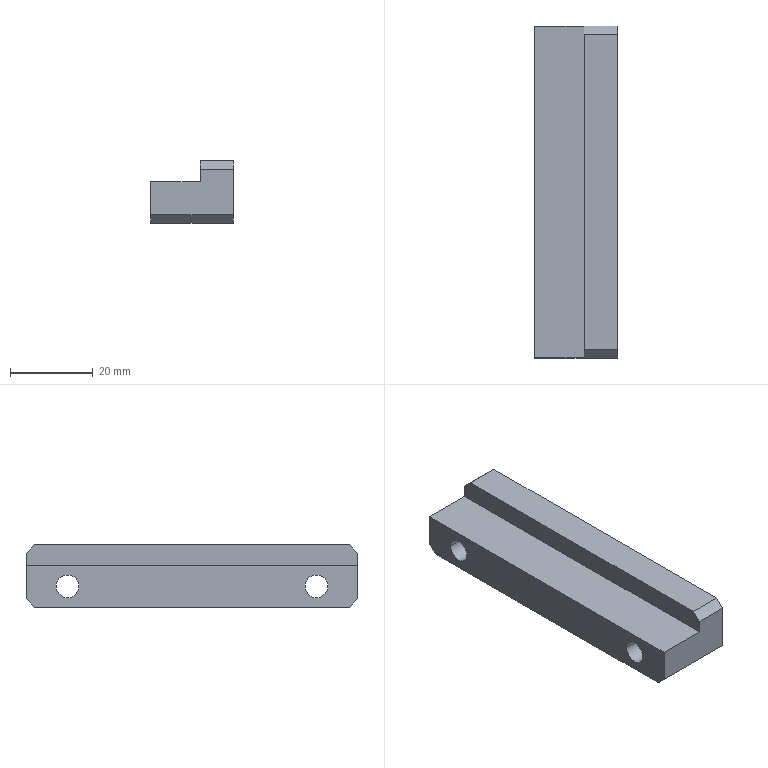Component | SolidWorks | ClampingAssembly-1_A84-2 | 1 solid | 24 faces | box 20 x 80 x 15 mm | volume 17417 mm3 | plane 18 | cylinder 6 | commonest cylinder face diameters 5.5 x4 10 x2 | material S136
build123d program:
from build123d import *

# Parameters (mm, degrees)
SKETCH1_W                  = 80
SKETCH1_H                  = 15
BOSS_EXTRUDE1_DEPTH        = 10
SKETCH2_W                  = 12
SKETCH2_H                  = 5
CUT_EXTRUDE1_DEPTH         = 81.971
CHAMFER1_SIZE              = 2
F_5_5_5_5_DIAMETER_HOLE1_D = 5.5
CUT_EXTRUDE2_DEPTH         = 5.5


with BuildPart() as part:
    # Sketch1 → Boss-Extrude1 (new, symmetric)
    with BuildSketch(Plane(origin=(0, 0, 0), x_dir=(0, 0, -1), z_dir=(1, 0, 0))):
        Rectangle(SKETCH1_W, SKETCH1_H)
    extrude(amount=BOSS_EXTRUDE1_DEPTH, both=True)

    # Sketch2 → Cut-Extrude1 (cut, through all)
    with BuildSketch(Plane(origin=(0, 0, -40), x_dir=(-1, 0, 0), z_dir=(0, 0, -1))):
        with Locations((4, -5)):
            Rectangle(SKETCH2_W, SKETCH2_H)
    extrude(amount=-CUT_EXTRUDE1_DEPTH, mode=Mode.SUBTRACT)

    # Chamfer1
    chamfer1_edges = [part.edges().sort_by_distance(p)[0] for p in [
        (6, -7.5, -40),
        (6, -7.5, 40),
        (0, 7.5, 40),
        (0, 7.5, -40),
    ]]
    chamfer(chamfer1_edges, length=CHAMFER1_SIZE)

    # 5.5 _5.5_ Diameter Hole1 (through all)
    with Locations(Plane(origin=(10, 0, 0), x_dir=(0, 0, -1), z_dir=(1, 0, 0))):
        with Locations((-30, 2.5), (30, 2.5)):
            Hole(F_5_5_5_5_DIAMETER_HOLE1_D / 2)

    # Sketch7 → Cut-Extrude2 (cut)
    with BuildSketch(Plane(origin=(10, 0, 0), x_dir=(0, 0, -1), z_dir=(1, 0, 0))):
        with BuildLine():
            Line((-35, 2.5), (-35, 7.5))
            ThreePointArc((-35, 7.5), (-30, 12.5), (-25, 7.5))
            Line((-25, 7.5), (-25, 2.5))
            ThreePointArc((-25, 2.5), (-30, -2.5), (-35, 2.5))
        make_face()
        with BuildLine():
            Line((25, 2.5), (25, 7.5))
            ThreePointArc((25, 7.5), (30, 12.5), (35, 7.5))
            Line((35, 7.5), (35, 2.5))
            ThreePointArc((35, 2.5), (30, -2.5), (25, 2.5))
        make_face()
    extrude(amount=-CUT_EXTRUDE2_DEPTH, mode=Mode.SUBTRACT)


solid = part.part

# Placed as in the assembly
solid = solid.moved(Location((-4.551, 48.036, -72), (-90, 0, 0)))
STEP:
#1=COLOUR_RGB('',0.7922,0.8196,0.9333);
#2=FILL_AREA_STYLE_COLOUR('',#1);
#3=FILL_AREA_STYLE('',(#2));
#4=SURFACE_STYLE_FILL_AREA(#3);
#5=SURFACE_SIDE_STYLE('',(#4));
#6=SURFACE_STYLE_USAGE(.BOTH.,#5);
#7=PRESENTATION_STYLE_ASSIGNMENT((#6));
#8=CARTESIAN_POINT('',(-0.5729,3.181,-2.933));
#9=VERTEX_POINT('',#8);
#10=CARTESIAN_POINT('',(-0.5729,2.964,-2.933));
#11=VERTEX_POINT('',#10);
#12=CARTESIAN_POINT('',(-0.5729,3.072,-2.933));
#13=DIRECTION('',(1.,-0.,-0.));
#14=DIRECTION('',(0.,-1.,0.));
#15=AXIS2_PLACEMENT_3D('',#12,#13,#14);
#16=CIRCLE('',#15,0.1083);
#17=EDGE_CURVE('',#9,#11,#16,.T.);
#18=ORIENTED_EDGE('',*,*,#17,.F.);
#19=CARTESIAN_POINT('',(-0.001999,3.181,-2.933));
#20=VERTEX_POINT('',#19);
#21=CARTESIAN_POINT('',(0.2145,3.181,-2.933));
#22=DIRECTION('',(1.,-0.,-0.));
#23=VECTOR('',#22,39.37);
#24=LINE('',#21,#23);
#25=EDGE_CURVE('',#9,#20,#24,.T.);
#26=ORIENTED_EDGE('',*,*,#25,.T.);
#27=CARTESIAN_POINT('',(-0.001999,2.964,-2.933));
#28=VERTEX_POINT('',#27);
#29=CARTESIAN_POINT('',(-0.001999,3.072,-2.933));
#30=DIRECTION('',(-1.,0.,0.));
#31=DIRECTION('',(-0.,-1.,0.));
#32=AXIS2_PLACEMENT_3D('',#29,#30,#31);
#33=CIRCLE('',#32,0.1083);
#34=EDGE_CURVE('',#28,#20,#33,.T.);
#35=ORIENTED_EDGE('',*,*,#34,.F.);
#36=CARTESIAN_POINT('',(0.2145,2.964,-2.933));
#37=DIRECTION('',(1.,-0.,-0.));
#38=VECTOR('',#37,39.37);
#39=LINE('',#36,#38);
#40=EDGE_CURVE('',#11,#28,#39,.T.);
#41=ORIENTED_EDGE('',*,*,#40,.F.);
#42=EDGE_LOOP('',(#18,#26,#35,#41));
#43=FACE_OUTER_BOUND('',#42,.T.);
#44=CARTESIAN_POINT('',(0.2145,3.072,-2.933));
#45=DIRECTION('',(1.,-0.,-0.));
#46=DIRECTION('',(0.,-1.,0.));
#47=AXIS2_PLACEMENT_3D('',#44,#45,#46);
#48=CYLINDRICAL_SURFACE('',#47,0.1083);
#49=ADVANCED_FACE('',(#43),#48,.F.);
#50=CARTESIAN_POINT('',(-0.5729,0.8183,-2.933));
#51=VERTEX_POINT('',#50);
#52=CARTESIAN_POINT('',(-0.5729,0.6018,-2.933));
#53=VERTEX_POINT('',#52);
#54=CARTESIAN_POINT('',(-0.5729,0.7101,-2.933));
#55=DIRECTION('',(1.,-0.,-0.));
#56=DIRECTION('',(0.,-1.,0.));
#57=AXIS2_PLACEMENT_3D('',#54,#55,#56);
#58=CIRCLE('',#57,0.1083);
#59=EDGE_CURVE('',#51,#53,#58,.T.);
#60=ORIENTED_EDGE('',*,*,#59,.F.);
#61=CARTESIAN_POINT('',(-0.001999,0.8183,-2.933));
#62=VERTEX_POINT('',#61);
#63=CARTESIAN_POINT('',(0.2145,0.8183,-2.933));
#64=DIRECTION('',(1.,-0.,-0.));
#65=VECTOR('',#64,39.37);
#66=LINE('',#63,#65);
#67=EDGE_CURVE('',#51,#62,#66,.T.);
#68=ORIENTED_EDGE('',*,*,#67,.T.);
#69=CARTESIAN_POINT('',(-0.001999,0.6018,-2.933));
#70=VERTEX_POINT('',#69);
#71=CARTESIAN_POINT('',(-0.001999,0.7101,-2.933));
#72=DIRECTION('',(-1.,0.,0.));
#73=DIRECTION('',(-0.,-1.,0.));
#74=AXIS2_PLACEMENT_3D('',#71,#72,#73);
#75=CIRCLE('',#74,0.1083);
#76=EDGE_CURVE('',#70,#62,#75,.T.);
#77=ORIENTED_EDGE('',*,*,#76,.F.);
#78=CARTESIAN_POINT('',(0.2145,0.6018,-2.933));
#79=DIRECTION('',(1.,-0.,-0.));
#80=VECTOR('',#79,39.37);
#81=LINE('',#78,#80);
#82=EDGE_CURVE('',#53,#70,#81,.T.);
#83=ORIENTED_EDGE('',*,*,#82,.F.);
#84=EDGE_LOOP('',(#60,#68,#77,#83));
#85=FACE_OUTER_BOUND('',#84,.T.);
#86=CARTESIAN_POINT('',(0.2145,0.7101,-2.933));
#87=DIRECTION('',(1.,-0.,-0.));
#88=DIRECTION('',(0.,-1.,0.));
#89=AXIS2_PLACEMENT_3D('',#86,#87,#88);
#90=CYLINDRICAL_SURFACE('',#89,0.1083);
#91=ADVANCED_FACE('',(#85),#90,.F.);
#92=ORIENTED_EDGE('',*,*,#67,.F.);
#93=CARTESIAN_POINT('',(-0.5729,0.7101,-2.933));
#94=DIRECTION('',(1.,-0.,-0.));
#95=DIRECTION('',(0.,-1.,0.));
#96=AXIS2_PLACEMENT_3D('',#93,#94,#95);
#97=CIRCLE('',#96,0.1083);
#98=EDGE_CURVE('',#53,#51,#97,.T.);
#99=ORIENTED_EDGE('',*,*,#98,.F.);
#100=ORIENTED_EDGE('',*,*,#82,.T.);
#101=CARTESIAN_POINT('',(-0.001999,0.7101,-2.933));
#102=DIRECTION('',(-1.,0.,0.));
#103=DIRECTION('',(-0.,-1.,0.));
#104=AXIS2_PLACEMENT_3D('',#101,#102,#103);
#105=CIRCLE('',#104,0.1083);
#106=EDGE_CURVE('',#62,#70,#105,.T.);
#107=ORIENTED_EDGE('',*,*,#106,.F.);
#108=EDGE_LOOP('',(#92,#99,#100,#107));
#109=FACE_OUTER_BOUND('',#108,.T.);
#110=CARTESIAN_POINT('',(0.2145,0.7101,-2.933));
#111=DIRECTION('',(1.,-0.,-0.));
#112=DIRECTION('',(0.,-1.,0.));
#113=AXIS2_PLACEMENT_3D('',#110,#111,#112);
#114=CYLINDRICAL_SURFACE('',#113,0.1083);
#115=ADVANCED_FACE('',(#109),#114,.F.);
#116=ORIENTED_EDGE('',*,*,#25,.F.);
#117=CARTESIAN_POINT('',(-0.5729,3.072,-2.933));
#118=DIRECTION('',(1.,-0.,-0.));
#119=DIRECTION('',(0.,-1.,0.));
#120=AXIS2_PLACEMENT_3D('',#117,#118,#119);
#121=CIRCLE('',#120,0.1083);
#122=EDGE_CURVE('',#11,#9,#121,.T.);
#123=ORIENTED_EDGE('',*,*,#122,.F.);
#124=ORIENTED_EDGE('',*,*,#40,.T.);
#125=CARTESIAN_POINT('',(-0.001999,3.072,-2.933));
#126=DIRECTION('',(-1.,0.,0.));
#127=DIRECTION('',(-0.,-1.,0.));
#128=AXIS2_PLACEMENT_3D('',#125,#126,#127);
#129=CIRCLE('',#128,0.1083);
#130=EDGE_CURVE('',#20,#28,#129,.T.);
#131=ORIENTED_EDGE('',*,*,#130,.F.);
#132=EDGE_LOOP('',(#116,#123,#124,#131));
#133=FACE_OUTER_BOUND('',#132,.T.);
#134=CARTESIAN_POINT('',(0.2145,3.072,-2.933));
#135=DIRECTION('',(1.,-0.,-0.));
#136=DIRECTION('',(0.,-1.,0.));
#137=AXIS2_PLACEMENT_3D('',#134,#135,#136);
#138=CYLINDRICAL_SURFACE('',#137,0.1083);
#139=ADVANCED_FACE('',(#133),#138,.F.);
#140=CARTESIAN_POINT('',(-0.5729,0.3164,-2.736));
#141=VERTEX_POINT('',#140);
#142=CARTESIAN_POINT('',(-0.5729,0.3164,-3.051));
#143=VERTEX_POINT('',#142);
#144=CARTESIAN_POINT('',(-0.5729,0.3164,-3.13));
#145=DIRECTION('',(-0.,0.,-1.));
#146=VECTOR('',#145,39.37);
#147=LINE('',#144,#146);
#148=EDGE_CURVE('',#141,#143,#147,.T.);
#149=ORIENTED_EDGE('',*,*,#148,.T.);
#150=CARTESIAN_POINT('',(0.2145,0.3164,-3.051));
#151=VERTEX_POINT('',#150);
#152=CARTESIAN_POINT('',(0.2145,0.3164,-3.051));
#153=DIRECTION('',(1.,-0.,-0.));
#154=VECTOR('',#153,39.37);
#155=LINE('',#152,#154);
#156=EDGE_CURVE('',#143,#151,#155,.T.);
#157=ORIENTED_EDGE('',*,*,#156,.T.);
#158=CARTESIAN_POINT('',(0.2145,0.3164,-2.618));
#159=VERTEX_POINT('',#158);
#160=CARTESIAN_POINT('',(0.2145,0.3164,-3.13));
#161=DIRECTION('',(-0.,0.,-1.));
#162=VECTOR('',#161,39.37);
#163=LINE('',#160,#162);
#164=EDGE_CURVE('',#159,#151,#163,.T.);
#165=ORIENTED_EDGE('',*,*,#164,.F.);
#166=CARTESIAN_POINT('',(-0.1004,0.3164,-2.618));
#167=VERTEX_POINT('',#166);
#168=CARTESIAN_POINT('',(0.2145,0.3164,-2.618));
#169=DIRECTION('',(-1.,0.,0.));
#170=VECTOR('',#169,39.37);
#171=LINE('',#168,#170);
#172=EDGE_CURVE('',#159,#167,#171,.T.);
#173=ORIENTED_EDGE('',*,*,#172,.T.);
#174=CARTESIAN_POINT('',(-0.1004,0.3164,-2.736));
#175=VERTEX_POINT('',#174);
#176=CARTESIAN_POINT('',(-0.1004,0.3164,-2.539));
#177=DIRECTION('',(0.,-0.,1.));
#178=VECTOR('',#177,39.37);
#179=LINE('',#176,#178);
#180=EDGE_CURVE('',#175,#167,#179,.T.);
#181=ORIENTED_EDGE('',*,*,#180,.F.);
#182=CARTESIAN_POINT('',(-0.5729,0.3164,-2.736));
#183=DIRECTION('',(1.,-0.,-0.));
#184=VECTOR('',#183,39.37);
#185=LINE('',#182,#184);
#186=EDGE_CURVE('',#141,#175,#185,.T.);
#187=ORIENTED_EDGE('',*,*,#186,.F.);
#188=EDGE_LOOP('',(#149,#157,#165,#173,#181,#187));
#189=FACE_OUTER_BOUND('',#188,.T.);
#190=CARTESIAN_POINT('',(0.2145,0.3164,-3.13));
#191=DIRECTION('',(0.,1.,0.));
#192=DIRECTION('',(0.,-0.,1.));
#193=AXIS2_PLACEMENT_3D('',#190,#191,#192);
#194=PLANE('',#193);
#195=ADVANCED_FACE('',(#189),#194,.F.);
#196=CARTESIAN_POINT('',(0.2145,3.269,-3.13));
#197=VERTEX_POINT('',#196);
#198=CARTESIAN_POINT('',(0.2145,3.387,-3.13));
#199=VERTEX_POINT('',#198);
#200=CARTESIAN_POINT('',(0.2145,3.466,-3.13));
#201=DIRECTION('',(0.,1.,0.));
#202=VECTOR('',#201,39.37);
#203=LINE('',#200,#202);
#204=EDGE_CURVE('',#197,#199,#203,.T.);
#205=ORIENTED_EDGE('',*,*,#204,.F.);
#206=CARTESIAN_POINT('',(-0.001999,3.269,-3.13));
#207=VERTEX_POINT('',#206);
#208=CARTESIAN_POINT('',(-0.001999,3.269,-3.13));
#209=DIRECTION('',(1.,-0.,-0.));
#210=VECTOR('',#209,39.37);
#211=LINE('',#208,#210);
#212=EDGE_CURVE('',#207,#197,#211,.T.);
#213=ORIENTED_EDGE('',*,*,#212,.F.);
#214=CARTESIAN_POINT('',(-0.001999,2.875,-3.13));
#215=VERTEX_POINT('',#214);
#216=CARTESIAN_POINT('',(-0.001999,3.466,-3.13));
#217=DIRECTION('',(0.,1.,0.));
#218=VECTOR('',#217,39.37);
#219=LINE('',#216,#218);
#220=EDGE_CURVE('',#215,#207,#219,.T.);
#221=ORIENTED_EDGE('',*,*,#220,.F.);
#222=CARTESIAN_POINT('',(0.2145,2.875,-3.13));
#223=VERTEX_POINT('',#222);
#224=CARTESIAN_POINT('',(-0.001999,2.875,-3.13));
#225=DIRECTION('',(1.,-0.,-0.));
#226=VECTOR('',#225,39.37);
#227=LINE('',#224,#226);
#228=EDGE_CURVE('',#215,#223,#227,.T.);
#229=ORIENTED_EDGE('',*,*,#228,.T.);
#230=CARTESIAN_POINT('',(0.2145,0.9069,-3.13));
#231=VERTEX_POINT('',#230);
#232=CARTESIAN_POINT('',(0.2145,3.466,-3.13));
#233=DIRECTION('',(0.,1.,0.));
#234=VECTOR('',#233,39.37);
#235=LINE('',#232,#234);
#236=EDGE_CURVE('',#231,#223,#235,.T.);
#237=ORIENTED_EDGE('',*,*,#236,.F.);
#238=CARTESIAN_POINT('',(-0.001999,0.9069,-3.13));
#239=VERTEX_POINT('',#238);
#240=CARTESIAN_POINT('',(-0.001999,0.9069,-3.13));
#241=DIRECTION('',(1.,-0.,-0.));
#242=VECTOR('',#241,39.37);
#243=LINE('',#240,#242);
#244=EDGE_CURVE('',#239,#231,#243,.T.);
#245=ORIENTED_EDGE('',*,*,#244,.F.);
#246=CARTESIAN_POINT('',(-0.001999,0.5132,-3.13));
#247=VERTEX_POINT('',#246);
#248=CARTESIAN_POINT('',(-0.001999,3.466,-3.13));
#249=DIRECTION('',(0.,1.,0.));
#250=VECTOR('',#249,39.37);
#251=LINE('',#248,#250);
#252=EDGE_CURVE('',#247,#239,#251,.T.);
#253=ORIENTED_EDGE('',*,*,#252,.F.);
#254=CARTESIAN_POINT('',(0.2145,0.5132,-3.13));
#255=VERTEX_POINT('',#254);
#256=CARTESIAN_POINT('',(-0.001999,0.5132,-3.13));
#257=DIRECTION('',(1.,-0.,-0.));
#258=VECTOR('',#257,39.37);
#259=LINE('',#256,#258);
#260=EDGE_CURVE('',#247,#255,#259,.T.);
#261=ORIENTED_EDGE('',*,*,#260,.T.);
#262=CARTESIAN_POINT('',(0.2145,0.3951,-3.13));
#263=VERTEX_POINT('',#262);
#264=CARTESIAN_POINT('',(0.2145,3.466,-3.13));
#265=DIRECTION('',(0.,1.,0.));
#266=VECTOR('',#265,39.37);
#267=LINE('',#264,#266);
#268=EDGE_CURVE('',#263,#255,#267,.T.);
#269=ORIENTED_EDGE('',*,*,#268,.F.);
#270=CARTESIAN_POINT('',(-0.5729,0.3951,-3.13));
#271=VERTEX_POINT('',#270);
#272=CARTESIAN_POINT('',(0.2145,0.3951,-3.13));
#273=DIRECTION('',(-1.,0.,0.));
#274=VECTOR('',#273,39.37);
#275=LINE('',#272,#274);
#276=EDGE_CURVE('',#263,#271,#275,.T.);
#277=ORIENTED_EDGE('',*,*,#276,.T.);
#278=CARTESIAN_POINT('',(-0.5729,3.387,-3.13));
#279=VERTEX_POINT('',#278);
#280=CARTESIAN_POINT('',(-0.5729,3.466,-3.13));
#281=DIRECTION('',(0.,1.,0.));
#282=VECTOR('',#281,39.37);
#283=LINE('',#280,#282);
#284=EDGE_CURVE('',#271,#279,#283,.T.);
#285=ORIENTED_EDGE('',*,*,#284,.T.);
#286=CARTESIAN_POINT('',(0.2145,3.387,-3.13));
#287=DIRECTION('',(1.,-0.,-0.));
#288=VECTOR('',#287,39.37);
#289=LINE('',#286,#288);
#290=EDGE_CURVE('',#279,#199,#289,.T.);
#291=ORIENTED_EDGE('',*,*,#290,.T.);
#292=EDGE_LOOP('',(#205,#213,#221,#229,#237,#245,#253,#261,#269,#277,#285,#291));
#293=FACE_OUTER_BOUND('',#292,.T.);
#294=CARTESIAN_POINT('',(0.2145,3.466,-3.13));
#295=DIRECTION('',(0.,-0.,1.));
#296=DIRECTION('',(-0.,-1.,-0.));
#297=AXIS2_PLACEMENT_3D('',#294,#295,#296);
#298=PLANE('',#297);
#299=ADVANCED_FACE('',(#293),#298,.F.);
#300=CARTESIAN_POINT('',(0.2145,3.466,-3.051));
#301=VERTEX_POINT('',#300);
#302=CARTESIAN_POINT('',(0.2145,3.466,-2.618));
#303=VERTEX_POINT('',#302);
#304=CARTESIAN_POINT('',(0.2145,3.466,-3.13));
#305=DIRECTION('',(0.,0.,1.));
#306=VECTOR('',#305,39.37);
#307=LINE('',#304,#306);
#308=EDGE_CURVE('',#301,#303,#307,.T.);
#309=ORIENTED_EDGE('',*,*,#308,.F.);
#310=CARTESIAN_POINT('',(-0.5729,3.466,-3.051));
#311=VERTEX_POINT('',#310);
#312=CARTESIAN_POINT('',(0.2145,3.466,-3.051));
#313=DIRECTION('',(-1.,0.,0.));
#314=VECTOR('',#313,39.37);
#315=LINE('',#312,#314);
#316=EDGE_CURVE('',#301,#311,#315,.T.);
#317=ORIENTED_EDGE('',*,*,#316,.T.);
#318=CARTESIAN_POINT('',(-0.5729,3.466,-2.736));
#319=VERTEX_POINT('',#318);
#320=CARTESIAN_POINT('',(-0.5729,3.466,-3.13));
#321=DIRECTION('',(0.,0.,1.));
#322=VECTOR('',#321,39.37);
#323=LINE('',#320,#322);
#324=EDGE_CURVE('',#311,#319,#323,.T.);
#325=ORIENTED_EDGE('',*,*,#324,.T.);
#326=CARTESIAN_POINT('',(-0.1004,3.466,-2.736));
#327=VERTEX_POINT('',#326);
#328=CARTESIAN_POINT('',(-0.5729,3.466,-2.736));
#329=DIRECTION('',(1.,-0.,-0.));
#330=VECTOR('',#329,39.37);
#331=LINE('',#328,#330);
#332=EDGE_CURVE('',#319,#327,#331,.T.);
#333=ORIENTED_EDGE('',*,*,#332,.T.);
#334=CARTESIAN_POINT('',(-0.1004,3.466,-2.618));
#335=VERTEX_POINT('',#334);
#336=CARTESIAN_POINT('',(-0.1004,3.466,-2.539));
#337=DIRECTION('',(0.,-0.,1.));
#338=VECTOR('',#337,39.37);
#339=LINE('',#336,#338);
#340=EDGE_CURVE('',#327,#335,#339,.T.);
#341=ORIENTED_EDGE('',*,*,#340,.T.);
#342=CARTESIAN_POINT('',(0.2145,3.466,-2.618));
#343=DIRECTION('',(1.,-0.,-0.));
#344=VECTOR('',#343,39.37);
#345=LINE('',#342,#344);
#346=EDGE_CURVE('',#335,#303,#345,.T.);
#347=ORIENTED_EDGE('',*,*,#346,.T.);
#348=EDGE_LOOP('',(#309,#317,#325,#333,#341,#347));
#349=FACE_OUTER_BOUND('',#348,.T.);
#350=CARTESIAN_POINT('',(0.2145,3.466,-3.13));
#351=DIRECTION('',(-0.,-1.,0.));
#352=DIRECTION('',(-0.,-0.,-1.));
#353=AXIS2_PLACEMENT_3D('',#350,#351,#352);
#354=PLANE('',#353);
#355=ADVANCED_FACE('',(#349),#354,.F.);
#356=CARTESIAN_POINT('',(0.2145,3.387,-2.539));
#357=VERTEX_POINT('',#356);
#358=CARTESIAN_POINT('',(0.2145,0.3951,-2.539));
#359=VERTEX_POINT('',#358);
#360=CARTESIAN_POINT('',(0.2145,3.466,-2.539));
#361=DIRECTION('',(-0.,-1.,-0.));
#362=VECTOR('',#361,39.37);
#363=LINE('',#360,#362);
#364=EDGE_CURVE('',#357,#359,#363,.T.);
#365=ORIENTED_EDGE('',*,*,#364,.F.);
#366=CARTESIAN_POINT('',(-0.1004,3.387,-2.539));
#367=VERTEX_POINT('',#366);
#368=CARTESIAN_POINT('',(0.2145,3.387,-2.539));
#369=DIRECTION('',(-1.,0.,0.));
#370=VECTOR('',#369,39.37);
#371=LINE('',#368,#370);
#372=EDGE_CURVE('',#357,#367,#371,.T.);
#373=ORIENTED_EDGE('',*,*,#372,.T.);
#374=CARTESIAN_POINT('',(-0.1004,0.3951,-2.539));
#375=VERTEX_POINT('',#374);
#376=CARTESIAN_POINT('',(-0.1004,3.466,-2.539));
#377=DIRECTION('',(-0.,-1.,-0.));
#378=VECTOR('',#377,39.37);
#379=LINE('',#376,#378);
#380=EDGE_CURVE('',#367,#375,#379,.T.);
#381=ORIENTED_EDGE('',*,*,#380,.T.);
#382=CARTESIAN_POINT('',(0.2145,0.3951,-2.539));
#383=DIRECTION('',(1.,-0.,-0.));
#384=VECTOR('',#383,39.37);
#385=LINE('',#382,#384);
#386=EDGE_CURVE('',#375,#359,#385,.T.);
#387=ORIENTED_EDGE('',*,*,#386,.T.);
#388=EDGE_LOOP('',(#365,#373,#381,#387));
#389=FACE_OUTER_BOUND('',#388,.T.);
#390=CARTESIAN_POINT('',(0.2145,3.466,-2.539));
#391=DIRECTION('',(-0.,0.,-1.));
#392=DIRECTION('',(0.,1.,0.));
#393=AXIS2_PLACEMENT_3D('',#390,#391,#392);
#394=PLANE('',#393);
#395=ADVANCED_FACE('',(#389),#394,.F.);
#396=CARTESIAN_POINT('',(0.2145,3.269,-2.933));
#397=VERTEX_POINT('',#396);
#398=CARTESIAN_POINT('',(0.2145,3.269,-2.933));
#399=DIRECTION('',(0.,-0.,1.));
#400=VECTOR('',#399,39.37);
#401=LINE('',#398,#400);
#402=EDGE_CURVE('',#197,#397,#401,.T.);
#403=ORIENTED_EDGE('',*,*,#402,.F.);
#404=ORIENTED_EDGE('',*,*,#204,.T.);
#405=CARTESIAN_POINT('',(0.2145,2.787,-3.73));
#406=DIRECTION('',(0.,0.7071,0.7071));
#407=VECTOR('',#406,39.37);
#408=LINE('',#405,#407);
#409=EDGE_CURVE('',#199,#301,#408,.T.);
#410=ORIENTED_EDGE('',*,*,#409,.T.);
#411=ORIENTED_EDGE('',*,*,#308,.T.);
#412=CARTESIAN_POINT('',(0.2145,2.787,-1.939));
#413=DIRECTION('',(0.,-0.7071,0.7071));
#414=VECTOR('',#413,39.37);
#415=LINE('',#412,#414);
#416=EDGE_CURVE('',#303,#357,#415,.T.);
#417=ORIENTED_EDGE('',*,*,#416,.T.);
#418=ORIENTED_EDGE('',*,*,#364,.T.);
#419=CARTESIAN_POINT('',(0.2145,0.9955,-1.939));
#420=DIRECTION('',(-0.,-0.7071,-0.7071));
#421=VECTOR('',#420,39.37);
#422=LINE('',#419,#421);
#423=EDGE_CURVE('',#359,#159,#422,.T.);
#424=ORIENTED_EDGE('',*,*,#423,.T.);
#425=ORIENTED_EDGE('',*,*,#164,.T.);
#426=CARTESIAN_POINT('',(0.2145,0.9955,-3.73));
#427=DIRECTION('',(-0.,0.7071,-0.7071));
#428=VECTOR('',#427,39.37);
#429=LINE('',#426,#428);
#430=EDGE_CURVE('',#151,#263,#429,.T.);
#431=ORIENTED_EDGE('',*,*,#430,.T.);
#432=ORIENTED_EDGE('',*,*,#268,.T.);
#433=CARTESIAN_POINT('',(0.2145,0.5132,-2.933));
#434=VERTEX_POINT('',#433);
#435=CARTESIAN_POINT('',(0.2145,0.5132,-2.933));
#436=DIRECTION('',(-0.,0.,-1.));
#437=VECTOR('',#436,39.37);
#438=LINE('',#435,#437);
#439=EDGE_CURVE('',#434,#255,#438,.T.);
#440=ORIENTED_EDGE('',*,*,#439,.F.);
#441=CARTESIAN_POINT('',(0.2145,0.9069,-2.933));
#442=VERTEX_POINT('',#441);
#443=CARTESIAN_POINT('',(0.2145,0.7101,-2.933));
#444=DIRECTION('',(1.,-0.,-0.));
#445=DIRECTION('',(0.,-1.,0.));
#446=AXIS2_PLACEMENT_3D('',#443,#444,#445);
#447=CIRCLE('',#446,0.1969);
#448=EDGE_CURVE('',#442,#434,#447,.T.);
#449=ORIENTED_EDGE('',*,*,#448,.F.);
#450=CARTESIAN_POINT('',(0.2145,0.9069,-2.933));
#451=DIRECTION('',(0.,-0.,1.));
#452=VECTOR('',#451,39.37);
#453=LINE('',#450,#452);
#454=EDGE_CURVE('',#231,#442,#453,.T.);
#455=ORIENTED_EDGE('',*,*,#454,.F.);
#456=ORIENTED_EDGE('',*,*,#236,.T.);
#457=CARTESIAN_POINT('',(0.2145,2.875,-2.933));
#458=VERTEX_POINT('',#457);
#459=CARTESIAN_POINT('',(0.2145,2.875,-2.933));
#460=DIRECTION('',(-0.,0.,-1.));
#461=VECTOR('',#460,39.37);
#462=LINE('',#459,#461);
#463=EDGE_CURVE('',#458,#223,#462,.T.);
#464=ORIENTED_EDGE('',*,*,#463,.F.);
#465=CARTESIAN_POINT('',(0.2145,3.072,-2.933));
#466=DIRECTION('',(1.,-0.,-0.));
#467=DIRECTION('',(0.,-1.,0.));
#468=AXIS2_PLACEMENT_3D('',#465,#466,#467);
#469=CIRCLE('',#468,0.1969);
#470=EDGE_CURVE('',#397,#458,#469,.T.);
#471=ORIENTED_EDGE('',*,*,#470,.F.);
#472=EDGE_LOOP('',(#403,#404,#410,#411,#417,#418,#424,#425,#431,#432,#440,#449,#455,#456,#464,#471));
#473=FACE_OUTER_BOUND('',#472,.T.);
#474=CARTESIAN_POINT('',(0.2145,1.891,-2.835));
#475=DIRECTION('',(1.,-0.,-0.));
#476=DIRECTION('',(-0.,-1.,-0.));
#477=AXIS2_PLACEMENT_3D('',#474,#475,#476);
#478=PLANE('',#477);
#479=ADVANCED_FACE('',(#473),#478,.T.);
#480=ORIENTED_EDGE('',*,*,#122,.T.);
#481=ORIENTED_EDGE('',*,*,#17,.T.);
#482=EDGE_LOOP('',(#480,#481));
#483=FACE_BOUND('',#482,.T.);
#484=ORIENTED_EDGE('',*,*,#98,.T.);
#485=ORIENTED_EDGE('',*,*,#59,.T.);
#486=EDGE_LOOP('',(#484,#485));
#487=FACE_BOUND('',#486,.T.);
#488=ORIENTED_EDGE('',*,*,#284,.F.);
#489=CARTESIAN_POINT('',(-0.5729,0.3951,-3.13));
#490=DIRECTION('',(0.,-0.7071,0.7071));
#491=VECTOR('',#490,39.37);
#492=LINE('',#489,#491);
#493=EDGE_CURVE('',#271,#143,#492,.T.);
#494=ORIENTED_EDGE('',*,*,#493,.T.);
#495=ORIENTED_EDGE('',*,*,#148,.F.);
#496=CARTESIAN_POINT('',(-0.5729,3.466,-2.736));
#497=DIRECTION('',(-0.,-1.,-0.));
#498=VECTOR('',#497,39.37);
#499=LINE('',#496,#498);
#500=EDGE_CURVE('',#319,#141,#499,.T.);
#501=ORIENTED_EDGE('',*,*,#500,.F.);
#502=ORIENTED_EDGE('',*,*,#324,.F.);
#503=CARTESIAN_POINT('',(-0.5729,3.466,-3.051));
#504=DIRECTION('',(-0.,-0.7071,-0.7071));
#505=VECTOR('',#504,39.37);
#506=LINE('',#503,#505);
#507=EDGE_CURVE('',#311,#279,#506,.T.);
#508=ORIENTED_EDGE('',*,*,#507,.T.);
#509=EDGE_LOOP('',(#488,#494,#495,#501,#502,#508));
#510=FACE_OUTER_BOUND('',#509,.T.);
#511=CARTESIAN_POINT('',(-0.5729,1.891,-2.835));
#512=DIRECTION('',(1.,-0.,-0.));
#513=DIRECTION('',(-0.,-1.,-0.));
#514=AXIS2_PLACEMENT_3D('',#511,#512,#513);
#515=PLANE('',#514);
#516=ADVANCED_FACE('',(#483,#487,#510),#515,.F.);
#517=ORIENTED_EDGE('',*,*,#380,.F.);
#518=CARTESIAN_POINT('',(-0.1004,3.387,-2.539));
#519=DIRECTION('',(-0.,0.7071,-0.7071));
#520=VECTOR('',#519,39.37);
#521=LINE('',#518,#520);
#522=EDGE_CURVE('',#367,#335,#521,.T.);
#523=ORIENTED_EDGE('',*,*,#522,.T.);
#524=ORIENTED_EDGE('',*,*,#340,.F.);
#525=CARTESIAN_POINT('',(-0.1004,3.466,-2.736));
#526=DIRECTION('',(-0.,-1.,-0.));
#527=VECTOR('',#526,39.37);
#528=LINE('',#525,#527);
#529=EDGE_CURVE('',#327,#175,#528,.T.);
#530=ORIENTED_EDGE('',*,*,#529,.T.);
#531=ORIENTED_EDGE('',*,*,#180,.T.);
#532=CARTESIAN_POINT('',(-0.1004,0.3164,-2.618));
#533=DIRECTION('',(0.,0.7071,0.7071));
#534=VECTOR('',#533,39.37);
#535=LINE('',#532,#534);
#536=EDGE_CURVE('',#167,#375,#535,.T.);
#537=ORIENTED_EDGE('',*,*,#536,.T.);
#538=EDGE_LOOP('',(#517,#523,#524,#530,#531,#537));
#539=FACE_OUTER_BOUND('',#538,.T.);
#540=CARTESIAN_POINT('',(-0.1004,3.466,-2.539));
#541=DIRECTION('',(1.,-0.,-0.));
#542=DIRECTION('',(-0.,-1.,-0.));
#543=AXIS2_PLACEMENT_3D('',#540,#541,#542);
#544=PLANE('',#543);
#545=ADVANCED_FACE('',(#539),#544,.F.);
#546=ORIENTED_EDGE('',*,*,#186,.T.);
#547=ORIENTED_EDGE('',*,*,#529,.F.);
#548=ORIENTED_EDGE('',*,*,#332,.F.);
#549=ORIENTED_EDGE('',*,*,#500,.T.);
#550=EDGE_LOOP('',(#546,#547,#548,#549));
#551=FACE_OUTER_BOUND('',#550,.T.);
#552=CARTESIAN_POINT('',(-0.5729,3.466,-2.736));
#553=DIRECTION('',(-0.,0.,-1.));
#554=DIRECTION('',(0.,1.,0.));
#555=AXIS2_PLACEMENT_3D('',#552,#553,#554);
#556=PLANE('',#555);
#557=ADVANCED_FACE('',(#551),#556,.F.);
#558=ORIENTED_EDGE('',*,*,#430,.F.);
#559=ORIENTED_EDGE('',*,*,#156,.F.);
#560=ORIENTED_EDGE('',*,*,#493,.F.);
#561=ORIENTED_EDGE('',*,*,#276,.F.);
#562=EDGE_LOOP('',(#558,#559,#560,#561));
#563=FACE_OUTER_BOUND('',#562,.T.);
#564=CARTESIAN_POINT('',(0.2145,0.3951,-3.13));
#565=DIRECTION('',(0.,0.7071,0.7071));
#566=DIRECTION('',(-1.,0.,0.));
#567=AXIS2_PLACEMENT_3D('',#564,#565,#566);
#568=PLANE('',#567);
#569=ADVANCED_FACE('',(#563),#568,.F.);
#570=ORIENTED_EDGE('',*,*,#409,.F.);
#571=ORIENTED_EDGE('',*,*,#290,.F.);
#572=ORIENTED_EDGE('',*,*,#507,.F.);
#573=ORIENTED_EDGE('',*,*,#316,.F.);
#574=EDGE_LOOP('',(#570,#571,#572,#573));
#575=FACE_OUTER_BOUND('',#574,.T.);
#576=CARTESIAN_POINT('',(0.2145,3.466,-3.051));
#577=DIRECTION('',(0.,-0.7071,0.7071));
#578=DIRECTION('',(-1.,0.,0.));
#579=AXIS2_PLACEMENT_3D('',#576,#577,#578);
#580=PLANE('',#579);
#581=ADVANCED_FACE('',(#575),#580,.F.);
#582=ORIENTED_EDGE('',*,*,#416,.F.);
#583=ORIENTED_EDGE('',*,*,#346,.F.);
#584=ORIENTED_EDGE('',*,*,#522,.F.);
#585=ORIENTED_EDGE('',*,*,#372,.F.);
#586=EDGE_LOOP('',(#582,#583,#584,#585));
#587=FACE_OUTER_BOUND('',#586,.T.);
#588=CARTESIAN_POINT('',(0.2145,3.387,-2.539));
#589=DIRECTION('',(-0.,-0.7071,-0.7071));
#590=DIRECTION('',(-1.,0.,0.));
#591=AXIS2_PLACEMENT_3D('',#588,#589,#590);
#592=PLANE('',#591);
#593=ADVANCED_FACE('',(#587),#592,.F.);
#594=ORIENTED_EDGE('',*,*,#423,.F.);
#595=ORIENTED_EDGE('',*,*,#386,.F.);
#596=ORIENTED_EDGE('',*,*,#536,.F.);
#597=ORIENTED_EDGE('',*,*,#172,.F.);
#598=EDGE_LOOP('',(#594,#595,#596,#597));
#599=FACE_OUTER_BOUND('',#598,.T.);
#600=CARTESIAN_POINT('',(0.2145,0.3164,-2.618));
#601=DIRECTION('',(-0.,0.7071,-0.7071));
#602=DIRECTION('',(-1.,0.,0.));
#603=AXIS2_PLACEMENT_3D('',#600,#601,#602);
#604=PLANE('',#603);
#605=ADVANCED_FACE('',(#599),#604,.F.);
#606=ORIENTED_EDGE('',*,*,#34,.T.);
#607=ORIENTED_EDGE('',*,*,#130,.T.);
#608=EDGE_LOOP('',(#606,#607));
#609=FACE_BOUND('',#608,.T.);
#610=ORIENTED_EDGE('',*,*,#220,.T.);
#611=CARTESIAN_POINT('',(-0.001999,3.269,-2.933));
#612=VERTEX_POINT('',#611);
#613=CARTESIAN_POINT('',(-0.001999,3.269,-2.933));
#614=DIRECTION('',(0.,-0.,1.));
#615=VECTOR('',#614,39.37);
#616=LINE('',#613,#615);
#617=EDGE_CURVE('',#207,#612,#616,.T.);
#618=ORIENTED_EDGE('',*,*,#617,.T.);
#619=CARTESIAN_POINT('',(-0.001999,2.875,-2.933));
#620=VERTEX_POINT('',#619);
#621=CARTESIAN_POINT('',(-0.001999,3.072,-2.933));
#622=DIRECTION('',(1.,-0.,-0.));
#623=DIRECTION('',(-0.,-1.,0.));
#624=AXIS2_PLACEMENT_3D('',#621,#622,#623);
#625=CIRCLE('',#624,0.1969);
#626=EDGE_CURVE('',#612,#620,#625,.T.);
#627=ORIENTED_EDGE('',*,*,#626,.T.);
#628=CARTESIAN_POINT('',(-0.001999,2.875,-2.933));
#629=DIRECTION('',(-0.,0.,-1.));
#630=VECTOR('',#629,39.37);
#631=LINE('',#628,#630);
#632=EDGE_CURVE('',#620,#215,#631,.T.);
#633=ORIENTED_EDGE('',*,*,#632,.T.);
#634=EDGE_LOOP('',(#610,#618,#627,#633));
#635=FACE_OUTER_BOUND('',#634,.T.);
#636=CARTESIAN_POINT('',(-0.001999,3.072,-2.933));
#637=DIRECTION('',(1.,-0.,-0.));
#638=DIRECTION('',(-0.,-1.,-0.));
#639=AXIS2_PLACEMENT_3D('',#636,#637,#638);
#640=PLANE('',#639);
#641=ADVANCED_FACE('',(#609,#635),#640,.T.);
#642=ORIENTED_EDGE('',*,*,#470,.T.);
#643=CARTESIAN_POINT('',(-0.001999,2.875,-2.933));
#644=DIRECTION('',(1.,-0.,-0.));
#645=VECTOR('',#644,39.37);
#646=LINE('',#643,#645);
#647=EDGE_CURVE('',#620,#458,#646,.T.);
#648=ORIENTED_EDGE('',*,*,#647,.F.);
#649=ORIENTED_EDGE('',*,*,#626,.F.);
#650=CARTESIAN_POINT('',(-0.001999,3.269,-2.933));
#651=DIRECTION('',(1.,-0.,-0.));
#652=VECTOR('',#651,39.37);
#653=LINE('',#650,#652);
#654=EDGE_CURVE('',#612,#397,#653,.T.);
#655=ORIENTED_EDGE('',*,*,#654,.T.);
#656=EDGE_LOOP('',(#642,#648,#649,#655));
#657=FACE_OUTER_BOUND('',#656,.T.);
#658=CARTESIAN_POINT('',(-0.001999,3.072,-2.933));
#659=DIRECTION('',(1.,-0.,-0.));
#660=DIRECTION('',(-0.,-1.,0.));
#661=AXIS2_PLACEMENT_3D('',#658,#659,#660);
#662=CYLINDRICAL_SURFACE('',#661,0.1969);
#663=ADVANCED_FACE('',(#657),#662,.F.);
#664=ORIENTED_EDGE('',*,*,#402,.T.);
#665=ORIENTED_EDGE('',*,*,#654,.F.);
#666=ORIENTED_EDGE('',*,*,#617,.F.);
#667=ORIENTED_EDGE('',*,*,#212,.T.);
#668=EDGE_LOOP('',(#664,#665,#666,#667));
#669=FACE_OUTER_BOUND('',#668,.T.);
#670=CARTESIAN_POINT('',(-0.001999,3.269,-2.933));
#671=DIRECTION('',(0.,1.,0.));
#672=DIRECTION('',(1.,-0.,-0.));
#673=AXIS2_PLACEMENT_3D('',#670,#671,#672);
#674=PLANE('',#673);
#675=ADVANCED_FACE('',(#669),#674,.F.);
#676=ORIENTED_EDGE('',*,*,#463,.T.);
#677=ORIENTED_EDGE('',*,*,#228,.F.);
#678=ORIENTED_EDGE('',*,*,#632,.F.);
#679=ORIENTED_EDGE('',*,*,#647,.T.);
#680=EDGE_LOOP('',(#676,#677,#678,#679));
#681=FACE_OUTER_BOUND('',#680,.T.);
#682=CARTESIAN_POINT('',(-0.001999,2.875,-2.933));
#683=DIRECTION('',(-0.,-1.,-0.));
#684=DIRECTION('',(-1.,0.,0.));
#685=AXIS2_PLACEMENT_3D('',#682,#683,#684);
#686=PLANE('',#685);
#687=ADVANCED_FACE('',(#681),#686,.F.);
#688=ORIENTED_EDGE('',*,*,#76,.T.);
#689=ORIENTED_EDGE('',*,*,#106,.T.);
#690=EDGE_LOOP('',(#688,#689));
#691=FACE_BOUND('',#690,.T.);
#692=ORIENTED_EDGE('',*,*,#252,.T.);
#693=CARTESIAN_POINT('',(-0.001999,0.9069,-2.933));
#694=VERTEX_POINT('',#693);
#695=CARTESIAN_POINT('',(-0.001999,0.9069,-2.933));
#696=DIRECTION('',(0.,-0.,1.));
#697=VECTOR('',#696,39.37);
#698=LINE('',#695,#697);
#699=EDGE_CURVE('',#239,#694,#698,.T.);
#700=ORIENTED_EDGE('',*,*,#699,.T.);
#701=CARTESIAN_POINT('',(-0.001999,0.5132,-2.933));
#702=VERTEX_POINT('',#701);
#703=CARTESIAN_POINT('',(-0.001999,0.7101,-2.933));
#704=DIRECTION('',(1.,-0.,-0.));
#705=DIRECTION('',(-0.,-1.,0.));
#706=AXIS2_PLACEMENT_3D('',#703,#704,#705);
#707=CIRCLE('',#706,0.1969);
#708=EDGE_CURVE('',#694,#702,#707,.T.);
#709=ORIENTED_EDGE('',*,*,#708,.T.);
#710=CARTESIAN_POINT('',(-0.001999,0.5132,-2.933));
#711=DIRECTION('',(-0.,0.,-1.));
#712=VECTOR('',#711,39.37);
#713=LINE('',#710,#712);
#714=EDGE_CURVE('',#702,#247,#713,.T.);
#715=ORIENTED_EDGE('',*,*,#714,.T.);
#716=EDGE_LOOP('',(#692,#700,#709,#715));
#717=FACE_OUTER_BOUND('',#716,.T.);
#718=CARTESIAN_POINT('',(-0.001999,0.7101,-2.933));
#719=DIRECTION('',(1.,-0.,-0.));
#720=DIRECTION('',(-0.,-1.,-0.));
#721=AXIS2_PLACEMENT_3D('',#718,#719,#720);
#722=PLANE('',#721);
#723=ADVANCED_FACE('',(#691,#717),#722,.T.);
#724=ORIENTED_EDGE('',*,*,#448,.T.);
#725=CARTESIAN_POINT('',(-0.001999,0.5132,-2.933));
#726=DIRECTION('',(1.,-0.,-0.));
#727=VECTOR('',#726,39.37);
#728=LINE('',#725,#727);
#729=EDGE_CURVE('',#702,#434,#728,.T.);
#730=ORIENTED_EDGE('',*,*,#729,.F.);
#731=ORIENTED_EDGE('',*,*,#708,.F.);
#732=CARTESIAN_POINT('',(-0.001999,0.9069,-2.933));
#733=DIRECTION('',(1.,-0.,-0.));
#734=VECTOR('',#733,39.37);
#735=LINE('',#732,#734);
#736=EDGE_CURVE('',#694,#442,#735,.T.);
#737=ORIENTED_EDGE('',*,*,#736,.T.);
#738=EDGE_LOOP('',(#724,#730,#731,#737));
#739=FACE_OUTER_BOUND('',#738,.T.);
#740=CARTESIAN_POINT('',(-0.001999,0.7101,-2.933));
#741=DIRECTION('',(1.,-0.,-0.));
#742=DIRECTION('',(-0.,-1.,0.));
#743=AXIS2_PLACEMENT_3D('',#740,#741,#742);
#744=CYLINDRICAL_SURFACE('',#743,0.1969);
#745=ADVANCED_FACE('',(#739),#744,.F.);
#746=ORIENTED_EDGE('',*,*,#454,.T.);
#747=ORIENTED_EDGE('',*,*,#736,.F.);
#748=ORIENTED_EDGE('',*,*,#699,.F.);
#749=ORIENTED_EDGE('',*,*,#244,.T.);
#750=EDGE_LOOP('',(#746,#747,#748,#749));
#751=FACE_OUTER_BOUND('',#750,.T.);
#752=CARTESIAN_POINT('',(-0.001999,0.9069,-2.933));
#753=DIRECTION('',(0.,1.,0.));
#754=DIRECTION('',(1.,-0.,-0.));
#755=AXIS2_PLACEMENT_3D('',#752,#753,#754);
#756=PLANE('',#755);
#757=ADVANCED_FACE('',(#751),#756,.F.);
#758=ORIENTED_EDGE('',*,*,#439,.T.);
#759=ORIENTED_EDGE('',*,*,#260,.F.);
#760=ORIENTED_EDGE('',*,*,#714,.F.);
#761=ORIENTED_EDGE('',*,*,#729,.T.);
#762=EDGE_LOOP('',(#758,#759,#760,#761));
#763=FACE_OUTER_BOUND('',#762,.T.);
#764=CARTESIAN_POINT('',(-0.001999,0.5132,-2.933));
#765=DIRECTION('',(-0.,-1.,-0.));
#766=DIRECTION('',(-1.,0.,0.));
#767=AXIS2_PLACEMENT_3D('',#764,#765,#766);
#768=PLANE('',#767);
#769=ADVANCED_FACE('',(#763),#768,.F.);
#770=CLOSED_SHELL('',(#49,#91,#115,#139,#195,#299,#355,#395,#479,#516,#545,#557,#569,#581,#593,#605,#641,#663,#675,#687,#723,#745,#757,#769));
#771=MANIFOLD_SOLID_BREP('',#770);
#772=STYLED_ITEM('',(#7),#771);
#773=PRESENTATION_LAYER_ASSIGNMENT('','',(#772));
#774=(LENGTH_UNIT()NAMED_UNIT(*)SI_UNIT($,.METRE.));
#775=LENGTH_MEASURE_WITH_UNIT(LENGTH_MEASURE(0.0254),#774);
#776=DIMENSIONAL_EXPONENTS(1.,0.,0.,0.,0.,0.,0.);
#777=(CONVERSION_BASED_UNIT('',#775)LENGTH_UNIT()NAMED_UNIT(#776));
#778=UNCERTAINTY_MEASURE_WITH_UNIT(LENGTH_MEASURE(0.00001),#777,'','');
#779=(NAMED_UNIT(*)PLANE_ANGLE_UNIT()SI_UNIT($,.RADIAN.));
#780=(NAMED_UNIT(*)SI_UNIT($,.STERADIAN.)SOLID_ANGLE_UNIT());
#781=(GEOMETRIC_REPRESENTATION_CONTEXT(3)GLOBAL_UNCERTAINTY_ASSIGNED_CONTEXT((#778))GLOBAL_UNIT_ASSIGNED_CONTEXT((#777,#779,#780))REPRESENTATION_CONTEXT('',''));
#782=MECHANICAL_DESIGN_GEOMETRIC_PRESENTATION_REPRESENTATION('',(#772),#781);
#783=CARTESIAN_POINT('',(0.,0.,0.));
#784=DIRECTION('',(0.,0.,1.));
#785=DIRECTION('',(1.,0.,0.));
#786=AXIS2_PLACEMENT_3D('',#783,#784,#785);
#787=(LENGTH_UNIT()NAMED_UNIT(*)SI_UNIT($,.METRE.));
#788=LENGTH_MEASURE_WITH_UNIT(LENGTH_MEASURE(0.0254),#787);
#789=DIMENSIONAL_EXPONENTS(1.,0.,0.,0.,0.,0.,0.);
#790=(CONVERSION_BASED_UNIT('',#788)LENGTH_UNIT()NAMED_UNIT(#789));
#791=UNCERTAINTY_MEASURE_WITH_UNIT(LENGTH_MEASURE(0.00001),#790,'','');
#792=(NAMED_UNIT(*)PLANE_ANGLE_UNIT()SI_UNIT($,.RADIAN.));
#793=(NAMED_UNIT(*)SI_UNIT($,.STERADIAN.)SOLID_ANGLE_UNIT());
#794=(GEOMETRIC_REPRESENTATION_CONTEXT(3)GLOBAL_UNCERTAINTY_ASSIGNED_CONTEXT((#791))GLOBAL_UNIT_ASSIGNED_CONTEXT((#790,#792,#793))REPRESENTATION_CONTEXT('',''));
#795=ADVANCED_BREP_SHAPE_REPRESENTATION('',(#771,#786),#794);